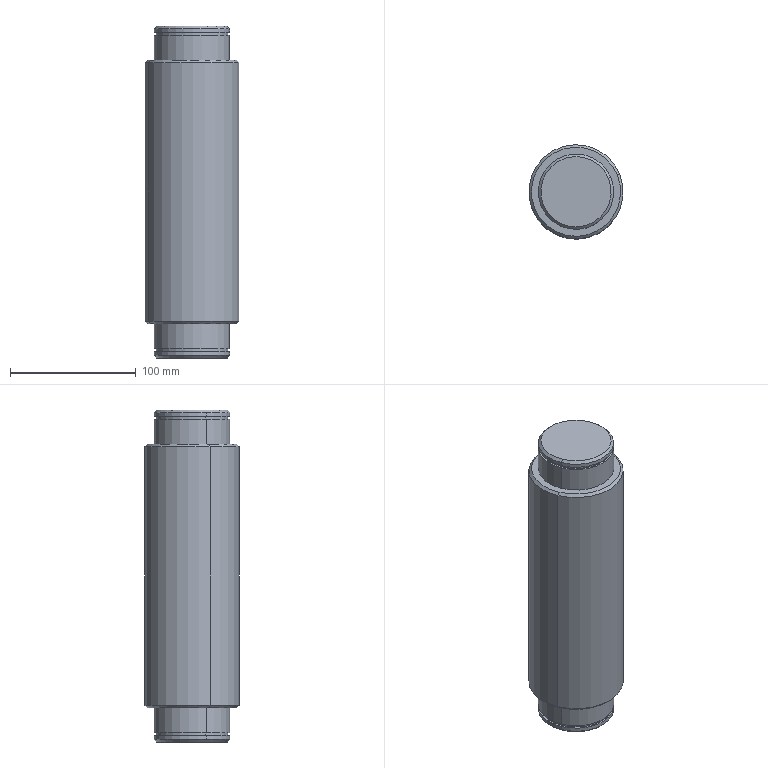Component | SolidWorks | RotationAxisB-1 | 1 solid | 30 faces | box 75 x 75 x 264.4 mm | volume 1078688 mm3 | cylinder 14 | cone 8 | plane 8 | commonest cylinder face diameters 60 x8 57 x4 75 x2 | material Stainless Steel
build123d program:
from build123d import *

# Parameters (mm, degrees)
CHAMFER1_SIZE = 2


with BuildPart() as part:
    # Sketch1 → Revolve1 (revolve)
    with BuildSketch(Plane.XY, mode=Mode.PRIVATE) as revolve1_sk:
        Polygon((0, 0), (0, 30), (5, 30), (5, 28.5), (7.2, 28.5), (7.2, 30), (27.2, 30), (27.2, 37.5), (237.2, 37.5), (237.2, 30), (257.2, 30), (257.2, 28.5), (259.4, 28.5), (259.4, 30), (264.4, 30), (264.4, 0), align=None)
    revolve(revolve1_sk.sketch.rotate(Axis((0, 0, 0), (1, 0, 0)), 90), axis=Axis((0, 0, 0), (1, 0, 0)))

    # Chamfer1
    chamfer1_edges = [part.edges().sort_by_distance(p)[0] for p in [
        (264.4, 0, -30),
        (237.2, 0, -37.5),
        (27.2, 0, -37.5),
        (0, 0, -30),
    ]]
    chamfer(chamfer1_edges, length=CHAMFER1_SIZE)


solid = part.part

# Placed as in the assembly
solid = solid.moved(Location((-534.67, 967.452, 382.9), (0, 90, 0)))
STEP:
#1=COLOUR_RGB('',0.7922,0.8196,0.9333);
#2=FILL_AREA_STYLE_COLOUR('',#1);
#3=FILL_AREA_STYLE('',(#2));
#4=SURFACE_STYLE_FILL_AREA(#3);
#5=SURFACE_SIDE_STYLE('',(#4));
#6=SURFACE_STYLE_USAGE(.BOTH.,#5);
#7=PRESENTATION_STYLE_ASSIGNMENT((#6));
#8=CARTESIAN_POINT('',(-22.068,37.666,15.075));
#9=VERTEX_POINT('',#8);
#10=CARTESIAN_POINT('',(-20.032,38.511,15.075));
#11=VERTEX_POINT('',#10);
#12=CARTESIAN_POINT('',(-21.05,38.089,15.075));
#13=DIRECTION('',(-0.,0.,1.));
#14=DIRECTION('',(0.9237,0.383,0.));
#15=AXIS2_PLACEMENT_3D('',#12,#13,#14);
#16=CIRCLE('',#15,1.102);
#17=EDGE_CURVE('',#9,#11,#16,.T.);
#18=ORIENTED_EDGE('',*,*,#17,.F.);
#19=CARTESIAN_POINT('',(-22.141,37.636,14.996));
#20=VERTEX_POINT('',#19);
#21=CARTESIAN_POINT('',(-22.068,37.666,15.075));
#22=DIRECTION('',(-0.6532,-0.2709,-0.7071));
#23=VECTOR('',#22,39.37);
#24=LINE('',#21,#23);
#25=EDGE_CURVE('',#9,#20,#24,.T.);
#26=ORIENTED_EDGE('',*,*,#25,.T.);
#27=CARTESIAN_POINT('',(-19.959,38.541,14.996));
#28=VERTEX_POINT('',#27);
#29=CARTESIAN_POINT('',(-21.05,38.089,14.996));
#30=DIRECTION('',(0.,-0.,-1.));
#31=DIRECTION('',(0.9237,0.383,0.));
#32=AXIS2_PLACEMENT_3D('',#29,#30,#31);
#33=CIRCLE('',#32,1.181);
#34=EDGE_CURVE('',#28,#20,#33,.T.);
#35=ORIENTED_EDGE('',*,*,#34,.F.);
#36=CARTESIAN_POINT('',(-20.032,38.511,15.075));
#37=DIRECTION('',(0.6532,0.2709,-0.7071));
#38=VECTOR('',#37,39.37);
#39=LINE('',#36,#38);
#40=EDGE_CURVE('',#11,#28,#39,.T.);
#41=ORIENTED_EDGE('',*,*,#40,.F.);
#42=EDGE_LOOP('',(#18,#26,#35,#41));
#43=FACE_OUTER_BOUND('',#42,.T.);
#44=CARTESIAN_POINT('',(-21.05,38.089,15.075));
#45=DIRECTION('',(0.,-0.,-1.));
#46=DIRECTION('',(0.9237,0.383,0.));
#47=AXIS2_PLACEMENT_3D('',#44,#45,#46);
#48=CONICAL_SURFACE('',#47,1.102,0.7854);
#49=ADVANCED_FACE('',(#43),#48,.T.);
#50=CARTESIAN_POINT('',(-22.341,37.553,14.004));
#51=VERTEX_POINT('',#50);
#52=CARTESIAN_POINT('',(-19.759,38.624,14.004));
#53=VERTEX_POINT('',#52);
#54=CARTESIAN_POINT('',(-21.05,38.089,14.004));
#55=DIRECTION('',(-0.,0.,1.));
#56=DIRECTION('',(0.9237,0.383,0.));
#57=AXIS2_PLACEMENT_3D('',#54,#55,#56);
#58=CIRCLE('',#57,1.398);
#59=EDGE_CURVE('',#51,#53,#58,.T.);
#60=ORIENTED_EDGE('',*,*,#59,.F.);
#61=CARTESIAN_POINT('',(-22.414,37.523,13.925));
#62=VERTEX_POINT('',#61);
#63=CARTESIAN_POINT('',(-22.341,37.553,14.004));
#64=DIRECTION('',(-0.6532,-0.2709,-0.7071));
#65=VECTOR('',#64,39.37);
#66=LINE('',#63,#65);
#67=EDGE_CURVE('',#51,#62,#66,.T.);
#68=ORIENTED_EDGE('',*,*,#67,.T.);
#69=CARTESIAN_POINT('',(-19.686,38.654,13.925));
#70=VERTEX_POINT('',#69);
#71=CARTESIAN_POINT('',(-21.05,38.089,13.925));
#72=DIRECTION('',(0.,-0.,-1.));
#73=DIRECTION('',(0.9237,0.383,0.));
#74=AXIS2_PLACEMENT_3D('',#71,#72,#73);
#75=CIRCLE('',#74,1.476);
#76=EDGE_CURVE('',#70,#62,#75,.T.);
#77=ORIENTED_EDGE('',*,*,#76,.F.);
#78=CARTESIAN_POINT('',(-19.759,38.624,14.004));
#79=DIRECTION('',(0.6532,0.2709,-0.7071));
#80=VECTOR('',#79,39.37);
#81=LINE('',#78,#80);
#82=EDGE_CURVE('',#53,#70,#81,.T.);
#83=ORIENTED_EDGE('',*,*,#82,.F.);
#84=EDGE_LOOP('',(#60,#68,#77,#83));
#85=FACE_OUTER_BOUND('',#84,.T.);
#86=CARTESIAN_POINT('',(-21.05,38.089,14.004));
#87=DIRECTION('',(0.,-0.,-1.));
#88=DIRECTION('',(0.9237,0.383,0.));
#89=AXIS2_PLACEMENT_3D('',#86,#87,#88);
#90=CONICAL_SURFACE('',#89,1.398,0.7854);
#91=ADVANCED_FACE('',(#85),#90,.T.);
#92=CARTESIAN_POINT('',(-19.759,38.624,5.736));
#93=VERTEX_POINT('',#92);
#94=CARTESIAN_POINT('',(-22.341,37.553,5.736));
#95=VERTEX_POINT('',#94);
#96=CARTESIAN_POINT('',(-21.05,38.089,5.736));
#97=DIRECTION('',(0.,-0.,-1.));
#98=DIRECTION('',(-0.9237,-0.383,0.));
#99=AXIS2_PLACEMENT_3D('',#96,#97,#98);
#100=CIRCLE('',#99,1.398);
#101=EDGE_CURVE('',#93,#95,#100,.T.);
#102=ORIENTED_EDGE('',*,*,#101,.F.);
#103=CARTESIAN_POINT('',(-19.686,38.654,5.815));
#104=VERTEX_POINT('',#103);
#105=CARTESIAN_POINT('',(-19.686,38.654,5.815));
#106=DIRECTION('',(0.6532,0.2709,0.7071));
#107=VECTOR('',#106,39.37);
#108=LINE('',#105,#107);
#109=EDGE_CURVE('',#93,#104,#108,.T.);
#110=ORIENTED_EDGE('',*,*,#109,.T.);
#111=CARTESIAN_POINT('',(-22.414,37.523,5.815));
#112=VERTEX_POINT('',#111);
#113=CARTESIAN_POINT('',(-21.05,38.089,5.815));
#114=DIRECTION('',(-0.,0.,1.));
#115=DIRECTION('',(-0.9237,-0.383,0.));
#116=AXIS2_PLACEMENT_3D('',#113,#114,#115);
#117=CIRCLE('',#116,1.476);
#118=EDGE_CURVE('',#112,#104,#117,.T.);
#119=ORIENTED_EDGE('',*,*,#118,.F.);
#120=CARTESIAN_POINT('',(-22.414,37.523,5.815));
#121=DIRECTION('',(-0.6532,-0.2709,0.7071));
#122=VECTOR('',#121,39.37);
#123=LINE('',#120,#122);
#124=EDGE_CURVE('',#95,#112,#123,.T.);
#125=ORIENTED_EDGE('',*,*,#124,.F.);
#126=EDGE_LOOP('',(#102,#110,#119,#125));
#127=FACE_OUTER_BOUND('',#126,.T.);
#128=CARTESIAN_POINT('',(-21.05,38.089,5.815));
#129=DIRECTION('',(-0.,0.,1.));
#130=DIRECTION('',(-0.9237,-0.383,0.));
#131=AXIS2_PLACEMENT_3D('',#128,#129,#130);
#132=CONICAL_SURFACE('',#131,1.476,0.7854);
#133=ADVANCED_FACE('',(#127),#132,.T.);
#134=CARTESIAN_POINT('',(-20.032,38.511,4.665));
#135=VERTEX_POINT('',#134);
#136=CARTESIAN_POINT('',(-22.068,37.666,4.665));
#137=VERTEX_POINT('',#136);
#138=CARTESIAN_POINT('',(-21.05,38.089,4.665));
#139=DIRECTION('',(0.,-0.,-1.));
#140=DIRECTION('',(-0.9237,-0.383,0.));
#141=AXIS2_PLACEMENT_3D('',#138,#139,#140);
#142=CIRCLE('',#141,1.102);
#143=EDGE_CURVE('',#135,#137,#142,.T.);
#144=ORIENTED_EDGE('',*,*,#143,.F.);
#145=CARTESIAN_POINT('',(-19.959,38.541,4.744));
#146=VERTEX_POINT('',#145);
#147=CARTESIAN_POINT('',(-19.959,38.541,4.744));
#148=DIRECTION('',(0.6532,0.2709,0.7071));
#149=VECTOR('',#148,39.37);
#150=LINE('',#147,#149);
#151=EDGE_CURVE('',#135,#146,#150,.T.);
#152=ORIENTED_EDGE('',*,*,#151,.T.);
#153=CARTESIAN_POINT('',(-22.141,37.636,4.744));
#154=VERTEX_POINT('',#153);
#155=CARTESIAN_POINT('',(-21.05,38.089,4.744));
#156=DIRECTION('',(-0.,0.,1.));
#157=DIRECTION('',(-0.9237,-0.383,0.));
#158=AXIS2_PLACEMENT_3D('',#155,#156,#157);
#159=CIRCLE('',#158,1.181);
#160=EDGE_CURVE('',#154,#146,#159,.T.);
#161=ORIENTED_EDGE('',*,*,#160,.F.);
#162=CARTESIAN_POINT('',(-22.141,37.636,4.744));
#163=DIRECTION('',(-0.6532,-0.2709,0.7071));
#164=VECTOR('',#163,39.37);
#165=LINE('',#162,#164);
#166=EDGE_CURVE('',#137,#154,#165,.T.);
#167=ORIENTED_EDGE('',*,*,#166,.F.);
#168=EDGE_LOOP('',(#144,#152,#161,#167));
#169=FACE_OUTER_BOUND('',#168,.T.);
#170=CARTESIAN_POINT('',(-21.05,38.089,4.744));
#171=DIRECTION('',(-0.,0.,1.));
#172=DIRECTION('',(-0.9237,-0.383,0.));
#173=AXIS2_PLACEMENT_3D('',#170,#171,#172);
#174=CONICAL_SURFACE('',#173,1.181,0.7854);
#175=ADVANCED_FACE('',(#169),#174,.T.);
#176=ORIENTED_EDGE('',*,*,#160,.T.);
#177=CARTESIAN_POINT('',(-19.959,38.541,4.862));
#178=VERTEX_POINT('',#177);
#179=CARTESIAN_POINT('',(-19.959,38.541,15.075));
#180=DIRECTION('',(-0.,0.,1.));
#181=VECTOR('',#180,39.37);
#182=LINE('',#179,#181);
#183=EDGE_CURVE('',#146,#178,#182,.T.);
#184=ORIENTED_EDGE('',*,*,#183,.T.);
#185=CARTESIAN_POINT('',(-22.141,37.636,4.862));
#186=VERTEX_POINT('',#185);
#187=CARTESIAN_POINT('',(-21.05,38.089,4.862));
#188=DIRECTION('',(-0.,0.,1.));
#189=DIRECTION('',(-0.9237,-0.383,0.));
#190=AXIS2_PLACEMENT_3D('',#187,#188,#189);
#191=CIRCLE('',#190,1.181);
#192=EDGE_CURVE('',#186,#178,#191,.T.);
#193=ORIENTED_EDGE('',*,*,#192,.F.);
#194=CARTESIAN_POINT('',(-22.141,37.636,15.075));
#195=DIRECTION('',(-0.,0.,1.));
#196=VECTOR('',#195,39.37);
#197=LINE('',#194,#196);
#198=EDGE_CURVE('',#154,#186,#197,.T.);
#199=ORIENTED_EDGE('',*,*,#198,.F.);
#200=EDGE_LOOP('',(#176,#184,#193,#199));
#201=FACE_OUTER_BOUND('',#200,.T.);
#202=CARTESIAN_POINT('',(-21.05,38.089,15.075));
#203=DIRECTION('',(-0.,0.,1.));
#204=DIRECTION('',(-0.9237,-0.383,0.));
#205=AXIS2_PLACEMENT_3D('',#202,#203,#204);
#206=CYLINDRICAL_SURFACE('',#205,1.181);
#207=ADVANCED_FACE('',(#201),#206,.T.);
#208=CARTESIAN_POINT('',(-22.086,37.659,4.862));
#209=VERTEX_POINT('',#208);
#210=CARTESIAN_POINT('',(-20.014,38.518,4.862));
#211=VERTEX_POINT('',#210);
#212=CARTESIAN_POINT('',(-21.05,38.089,4.862));
#213=DIRECTION('',(-0.,0.,1.));
#214=DIRECTION('',(-0.9237,-0.383,0.));
#215=AXIS2_PLACEMENT_3D('',#212,#213,#214);
#216=CIRCLE('',#215,1.122);
#217=EDGE_CURVE('',#209,#211,#216,.T.);
#218=ORIENTED_EDGE('',*,*,#217,.T.);
#219=CARTESIAN_POINT('',(-20.014,38.518,4.949));
#220=VERTEX_POINT('',#219);
#221=CARTESIAN_POINT('',(-20.014,38.518,15.075));
#222=DIRECTION('',(-0.,0.,1.));
#223=VECTOR('',#222,39.37);
#224=LINE('',#221,#223);
#225=EDGE_CURVE('',#211,#220,#224,.T.);
#226=ORIENTED_EDGE('',*,*,#225,.T.);
#227=CARTESIAN_POINT('',(-22.086,37.659,4.949));
#228=VERTEX_POINT('',#227);
#229=CARTESIAN_POINT('',(-21.05,38.089,4.949));
#230=DIRECTION('',(-0.,0.,1.));
#231=DIRECTION('',(-0.9237,-0.383,0.));
#232=AXIS2_PLACEMENT_3D('',#229,#230,#231);
#233=CIRCLE('',#232,1.122);
#234=EDGE_CURVE('',#228,#220,#233,.T.);
#235=ORIENTED_EDGE('',*,*,#234,.F.);
#236=CARTESIAN_POINT('',(-22.086,37.659,15.075));
#237=DIRECTION('',(-0.,0.,1.));
#238=VECTOR('',#237,39.37);
#239=LINE('',#236,#238);
#240=EDGE_CURVE('',#209,#228,#239,.T.);
#241=ORIENTED_EDGE('',*,*,#240,.F.);
#242=EDGE_LOOP('',(#218,#226,#235,#241));
#243=FACE_OUTER_BOUND('',#242,.T.);
#244=CARTESIAN_POINT('',(-21.05,38.089,15.075));
#245=DIRECTION('',(-0.,0.,1.));
#246=DIRECTION('',(-0.9237,-0.383,0.));
#247=AXIS2_PLACEMENT_3D('',#244,#245,#246);
#248=CYLINDRICAL_SURFACE('',#247,1.122);
#249=ADVANCED_FACE('',(#243),#248,.T.);
#250=CARTESIAN_POINT('',(-22.141,37.636,4.949));
#251=VERTEX_POINT('',#250);
#252=CARTESIAN_POINT('',(-19.959,38.541,4.949));
#253=VERTEX_POINT('',#252);
#254=CARTESIAN_POINT('',(-21.05,38.089,4.949));
#255=DIRECTION('',(-0.,0.,1.));
#256=DIRECTION('',(-0.9237,-0.383,0.));
#257=AXIS2_PLACEMENT_3D('',#254,#255,#256);
#258=CIRCLE('',#257,1.181);
#259=EDGE_CURVE('',#251,#253,#258,.T.);
#260=ORIENTED_EDGE('',*,*,#259,.T.);
#261=CARTESIAN_POINT('',(-19.959,38.541,5.736));
#262=VERTEX_POINT('',#261);
#263=CARTESIAN_POINT('',(-19.959,38.541,15.075));
#264=DIRECTION('',(-0.,0.,1.));
#265=VECTOR('',#264,39.37);
#266=LINE('',#263,#265);
#267=EDGE_CURVE('',#253,#262,#266,.T.);
#268=ORIENTED_EDGE('',*,*,#267,.T.);
#269=CARTESIAN_POINT('',(-22.141,37.636,5.736));
#270=VERTEX_POINT('',#269);
#271=CARTESIAN_POINT('',(-21.05,38.089,5.736));
#272=DIRECTION('',(-0.,0.,1.));
#273=DIRECTION('',(-0.9237,-0.383,0.));
#274=AXIS2_PLACEMENT_3D('',#271,#272,#273);
#275=CIRCLE('',#274,1.181);
#276=EDGE_CURVE('',#270,#262,#275,.T.);
#277=ORIENTED_EDGE('',*,*,#276,.F.);
#278=CARTESIAN_POINT('',(-22.141,37.636,15.075));
#279=DIRECTION('',(-0.,0.,1.));
#280=VECTOR('',#279,39.37);
#281=LINE('',#278,#280);
#282=EDGE_CURVE('',#251,#270,#281,.T.);
#283=ORIENTED_EDGE('',*,*,#282,.F.);
#284=EDGE_LOOP('',(#260,#268,#277,#283));
#285=FACE_OUTER_BOUND('',#284,.T.);
#286=CARTESIAN_POINT('',(-21.05,38.089,15.075));
#287=DIRECTION('',(-0.,0.,1.));
#288=DIRECTION('',(-0.9237,-0.383,0.));
#289=AXIS2_PLACEMENT_3D('',#286,#287,#288);
#290=CYLINDRICAL_SURFACE('',#289,1.181);
#291=ADVANCED_FACE('',(#285),#290,.T.);
#292=ORIENTED_EDGE('',*,*,#118,.T.);
#293=CARTESIAN_POINT('',(-19.686,38.654,15.075));
#294=DIRECTION('',(-0.,0.,1.));
#295=VECTOR('',#294,39.37);
#296=LINE('',#293,#295);
#297=EDGE_CURVE('',#104,#70,#296,.T.);
#298=ORIENTED_EDGE('',*,*,#297,.T.);
#299=ORIENTED_EDGE('',*,*,#76,.T.);
#300=CARTESIAN_POINT('',(-22.414,37.523,15.075));
#301=DIRECTION('',(-0.,0.,1.));
#302=VECTOR('',#301,39.37);
#303=LINE('',#300,#302);
#304=EDGE_CURVE('',#112,#62,#303,.T.);
#305=ORIENTED_EDGE('',*,*,#304,.F.);
#306=EDGE_LOOP('',(#292,#298,#299,#305));
#307=FACE_OUTER_BOUND('',#306,.T.);
#308=CARTESIAN_POINT('',(-21.05,38.089,15.075));
#309=DIRECTION('',(-0.,0.,1.));
#310=DIRECTION('',(-0.9237,-0.383,0.));
#311=AXIS2_PLACEMENT_3D('',#308,#309,#310);
#312=CYLINDRICAL_SURFACE('',#311,1.476);
#313=ADVANCED_FACE('',(#307),#312,.T.);
#314=CARTESIAN_POINT('',(-22.141,37.636,14.004));
#315=VERTEX_POINT('',#314);
#316=CARTESIAN_POINT('',(-19.959,38.541,14.004));
#317=VERTEX_POINT('',#316);
#318=CARTESIAN_POINT('',(-21.05,38.089,14.004));
#319=DIRECTION('',(-0.,0.,1.));
#320=DIRECTION('',(-0.9237,-0.383,0.));
#321=AXIS2_PLACEMENT_3D('',#318,#319,#320);
#322=CIRCLE('',#321,1.181);
#323=EDGE_CURVE('',#315,#317,#322,.T.);
#324=ORIENTED_EDGE('',*,*,#323,.T.);
#325=CARTESIAN_POINT('',(-19.959,38.541,14.791));
#326=VERTEX_POINT('',#325);
#327=CARTESIAN_POINT('',(-19.959,38.541,15.075));
#328=DIRECTION('',(-0.,0.,1.));
#329=VECTOR('',#328,39.37);
#330=LINE('',#327,#329);
#331=EDGE_CURVE('',#317,#326,#330,.T.);
#332=ORIENTED_EDGE('',*,*,#331,.T.);
#333=CARTESIAN_POINT('',(-22.141,37.636,14.791));
#334=VERTEX_POINT('',#333);
#335=CARTESIAN_POINT('',(-21.05,38.089,14.791));
#336=DIRECTION('',(-0.,0.,1.));
#337=DIRECTION('',(-0.9237,-0.383,0.));
#338=AXIS2_PLACEMENT_3D('',#335,#336,#337);
#339=CIRCLE('',#338,1.181);
#340=EDGE_CURVE('',#334,#326,#339,.T.);
#341=ORIENTED_EDGE('',*,*,#340,.F.);
#342=CARTESIAN_POINT('',(-22.141,37.636,15.075));
#343=DIRECTION('',(-0.,0.,1.));
#344=VECTOR('',#343,39.37);
#345=LINE('',#342,#344);
#346=EDGE_CURVE('',#315,#334,#345,.T.);
#347=ORIENTED_EDGE('',*,*,#346,.F.);
#348=EDGE_LOOP('',(#324,#332,#341,#347));
#349=FACE_OUTER_BOUND('',#348,.T.);
#350=CARTESIAN_POINT('',(-21.05,38.089,15.075));
#351=DIRECTION('',(-0.,0.,1.));
#352=DIRECTION('',(-0.9237,-0.383,0.));
#353=AXIS2_PLACEMENT_3D('',#350,#351,#352);
#354=CYLINDRICAL_SURFACE('',#353,1.181);
#355=ADVANCED_FACE('',(#349),#354,.T.);
#356=CARTESIAN_POINT('',(-22.086,37.659,14.791));
#357=VERTEX_POINT('',#356);
#358=CARTESIAN_POINT('',(-20.014,38.518,14.791));
#359=VERTEX_POINT('',#358);
#360=CARTESIAN_POINT('',(-21.05,38.089,14.791));
#361=DIRECTION('',(-0.,0.,1.));
#362=DIRECTION('',(-0.9237,-0.383,0.));
#363=AXIS2_PLACEMENT_3D('',#360,#361,#362);
#364=CIRCLE('',#363,1.122);
#365=EDGE_CURVE('',#357,#359,#364,.T.);
#366=ORIENTED_EDGE('',*,*,#365,.T.);
#367=CARTESIAN_POINT('',(-20.014,38.518,14.878));
#368=VERTEX_POINT('',#367);
#369=CARTESIAN_POINT('',(-20.014,38.518,15.075));
#370=DIRECTION('',(-0.,0.,1.));
#371=VECTOR('',#370,39.37);
#372=LINE('',#369,#371);
#373=EDGE_CURVE('',#359,#368,#372,.T.);
#374=ORIENTED_EDGE('',*,*,#373,.T.);
#375=CARTESIAN_POINT('',(-22.086,37.659,14.878));
#376=VERTEX_POINT('',#375);
#377=CARTESIAN_POINT('',(-21.05,38.089,14.878));
#378=DIRECTION('',(-0.,0.,1.));
#379=DIRECTION('',(-0.9237,-0.383,0.));
#380=AXIS2_PLACEMENT_3D('',#377,#378,#379);
#381=CIRCLE('',#380,1.122);
#382=EDGE_CURVE('',#376,#368,#381,.T.);
#383=ORIENTED_EDGE('',*,*,#382,.F.);
#384=CARTESIAN_POINT('',(-22.086,37.659,15.075));
#385=DIRECTION('',(-0.,0.,1.));
#386=VECTOR('',#385,39.37);
#387=LINE('',#384,#386);
#388=EDGE_CURVE('',#357,#376,#387,.T.);
#389=ORIENTED_EDGE('',*,*,#388,.F.);
#390=EDGE_LOOP('',(#366,#374,#383,#389));
#391=FACE_OUTER_BOUND('',#390,.T.);
#392=CARTESIAN_POINT('',(-21.05,38.089,15.075));
#393=DIRECTION('',(-0.,0.,1.));
#394=DIRECTION('',(-0.9237,-0.383,0.));
#395=AXIS2_PLACEMENT_3D('',#392,#393,#394);
#396=CYLINDRICAL_SURFACE('',#395,1.122);
#397=ADVANCED_FACE('',(#391),#396,.T.);
#398=CARTESIAN_POINT('',(-22.141,37.636,14.878));
#399=VERTEX_POINT('',#398);
#400=CARTESIAN_POINT('',(-19.959,38.541,14.878));
#401=VERTEX_POINT('',#400);
#402=CARTESIAN_POINT('',(-21.05,38.089,14.878));
#403=DIRECTION('',(-0.,0.,1.));
#404=DIRECTION('',(-0.9237,-0.383,0.));
#405=AXIS2_PLACEMENT_3D('',#402,#403,#404);
#406=CIRCLE('',#405,1.181);
#407=EDGE_CURVE('',#399,#401,#406,.T.);
#408=ORIENTED_EDGE('',*,*,#407,.T.);
#409=CARTESIAN_POINT('',(-19.959,38.541,15.075));
#410=DIRECTION('',(-0.,0.,1.));
#411=VECTOR('',#410,39.37);
#412=LINE('',#409,#411);
#413=EDGE_CURVE('',#401,#28,#412,.T.);
#414=ORIENTED_EDGE('',*,*,#413,.T.);
#415=ORIENTED_EDGE('',*,*,#34,.T.);
#416=CARTESIAN_POINT('',(-22.141,37.636,15.075));
#417=DIRECTION('',(-0.,0.,1.));
#418=VECTOR('',#417,39.37);
#419=LINE('',#416,#418);
#420=EDGE_CURVE('',#399,#20,#419,.T.);
#421=ORIENTED_EDGE('',*,*,#420,.F.);
#422=EDGE_LOOP('',(#408,#414,#415,#421));
#423=FACE_OUTER_BOUND('',#422,.T.);
#424=CARTESIAN_POINT('',(-21.05,38.089,15.075));
#425=DIRECTION('',(-0.,0.,1.));
#426=DIRECTION('',(-0.9237,-0.383,0.));
#427=AXIS2_PLACEMENT_3D('',#424,#425,#426);
#428=CYLINDRICAL_SURFACE('',#427,1.181);
#429=ADVANCED_FACE('',(#423),#428,.T.);
#430=CARTESIAN_POINT('',(-21.05,38.089,15.075));
#431=DIRECTION('',(-0.,0.,1.));
#432=DIRECTION('',(0.9237,0.383,0.));
#433=AXIS2_PLACEMENT_3D('',#430,#431,#432);
#434=CIRCLE('',#433,1.102);
#435=EDGE_CURVE('',#11,#9,#434,.T.);
#436=ORIENTED_EDGE('',*,*,#435,.T.);
#437=ORIENTED_EDGE('',*,*,#17,.T.);
#438=EDGE_LOOP('',(#436,#437));
#439=FACE_OUTER_BOUND('',#438,.T.);
#440=CARTESIAN_POINT('',(-21.05,38.089,15.075));
#441=DIRECTION('',(0.,-0.,-1.));
#442=DIRECTION('',(0.9237,0.383,0.));
#443=AXIS2_PLACEMENT_3D('',#440,#441,#442);
#444=PLANE('',#443);
#445=ADVANCED_FACE('',(#439),#444,.F.);
#446=ORIENTED_EDGE('',*,*,#413,.F.);
#447=CARTESIAN_POINT('',(-21.05,38.089,14.878));
#448=DIRECTION('',(-0.,0.,1.));
#449=DIRECTION('',(-0.9237,-0.383,0.));
#450=AXIS2_PLACEMENT_3D('',#447,#448,#449);
#451=CIRCLE('',#450,1.181);
#452=EDGE_CURVE('',#401,#399,#451,.T.);
#453=ORIENTED_EDGE('',*,*,#452,.T.);
#454=ORIENTED_EDGE('',*,*,#420,.T.);
#455=CARTESIAN_POINT('',(-21.05,38.089,14.996));
#456=DIRECTION('',(0.,-0.,-1.));
#457=DIRECTION('',(0.9237,0.383,0.));
#458=AXIS2_PLACEMENT_3D('',#455,#456,#457);
#459=CIRCLE('',#458,1.181);
#460=EDGE_CURVE('',#20,#28,#459,.T.);
#461=ORIENTED_EDGE('',*,*,#460,.T.);
#462=EDGE_LOOP('',(#446,#453,#454,#461));
#463=FACE_OUTER_BOUND('',#462,.T.);
#464=CARTESIAN_POINT('',(-21.05,38.089,15.075));
#465=DIRECTION('',(-0.,0.,1.));
#466=DIRECTION('',(-0.9237,-0.383,0.));
#467=AXIS2_PLACEMENT_3D('',#464,#465,#466);
#468=CYLINDRICAL_SURFACE('',#467,1.181);
#469=ADVANCED_FACE('',(#463),#468,.T.);
#470=ORIENTED_EDGE('',*,*,#407,.F.);
#471=ORIENTED_EDGE('',*,*,#452,.F.);
#472=EDGE_LOOP('',(#470,#471));
#473=FACE_OUTER_BOUND('',#472,.T.);
#474=ORIENTED_EDGE('',*,*,#382,.T.);
#475=CARTESIAN_POINT('',(-21.05,38.089,14.878));
#476=DIRECTION('',(-0.,0.,1.));
#477=DIRECTION('',(-0.9237,-0.383,0.));
#478=AXIS2_PLACEMENT_3D('',#475,#476,#477);
#479=CIRCLE('',#478,1.122);
#480=EDGE_CURVE('',#368,#376,#479,.T.);
#481=ORIENTED_EDGE('',*,*,#480,.T.);
#482=EDGE_LOOP('',(#474,#481));
#483=FACE_BOUND('',#482,.T.);
#484=CARTESIAN_POINT('',(-20.598,36.998,14.878));
#485=DIRECTION('',(-0.,0.,1.));
#486=DIRECTION('',(-0.9237,-0.383,-0.));
#487=AXIS2_PLACEMENT_3D('',#484,#485,#486);
#488=PLANE('',#487);
#489=ADVANCED_FACE('',(#473,#483),#488,.F.);
#490=ORIENTED_EDGE('',*,*,#373,.F.);
#491=CARTESIAN_POINT('',(-21.05,38.089,14.791));
#492=DIRECTION('',(-0.,0.,1.));
#493=DIRECTION('',(-0.9237,-0.383,0.));
#494=AXIS2_PLACEMENT_3D('',#491,#492,#493);
#495=CIRCLE('',#494,1.122);
#496=EDGE_CURVE('',#359,#357,#495,.T.);
#497=ORIENTED_EDGE('',*,*,#496,.T.);
#498=ORIENTED_EDGE('',*,*,#388,.T.);
#499=ORIENTED_EDGE('',*,*,#480,.F.);
#500=EDGE_LOOP('',(#490,#497,#498,#499));
#501=FACE_OUTER_BOUND('',#500,.T.);
#502=CARTESIAN_POINT('',(-21.05,38.089,15.075));
#503=DIRECTION('',(-0.,0.,1.));
#504=DIRECTION('',(-0.9237,-0.383,0.));
#505=AXIS2_PLACEMENT_3D('',#502,#503,#504);
#506=CYLINDRICAL_SURFACE('',#505,1.122);
#507=ADVANCED_FACE('',(#501),#506,.T.);
#508=ORIENTED_EDGE('',*,*,#365,.F.);
#509=ORIENTED_EDGE('',*,*,#496,.F.);
#510=EDGE_LOOP('',(#508,#509));
#511=FACE_BOUND('',#510,.T.);
#512=ORIENTED_EDGE('',*,*,#340,.T.);
#513=CARTESIAN_POINT('',(-21.05,38.089,14.791));
#514=DIRECTION('',(-0.,0.,1.));
#515=DIRECTION('',(-0.9237,-0.383,0.));
#516=AXIS2_PLACEMENT_3D('',#513,#514,#515);
#517=CIRCLE('',#516,1.181);
#518=EDGE_CURVE('',#326,#334,#517,.T.);
#519=ORIENTED_EDGE('',*,*,#518,.T.);
#520=EDGE_LOOP('',(#512,#519));
#521=FACE_OUTER_BOUND('',#520,.T.);
#522=CARTESIAN_POINT('',(-20.62,37.052,14.791));
#523=DIRECTION('',(0.,-0.,-1.));
#524=DIRECTION('',(0.9237,0.383,0.));
#525=AXIS2_PLACEMENT_3D('',#522,#523,#524);
#526=PLANE('',#525);
#527=ADVANCED_FACE('',(#511,#521),#526,.F.);
#528=ORIENTED_EDGE('',*,*,#331,.F.);
#529=CARTESIAN_POINT('',(-21.05,38.089,14.004));
#530=DIRECTION('',(-0.,0.,1.));
#531=DIRECTION('',(-0.9237,-0.383,0.));
#532=AXIS2_PLACEMENT_3D('',#529,#530,#531);
#533=CIRCLE('',#532,1.181);
#534=EDGE_CURVE('',#317,#315,#533,.T.);
#535=ORIENTED_EDGE('',*,*,#534,.T.);
#536=ORIENTED_EDGE('',*,*,#346,.T.);
#537=ORIENTED_EDGE('',*,*,#518,.F.);
#538=EDGE_LOOP('',(#528,#535,#536,#537));
#539=FACE_OUTER_BOUND('',#538,.T.);
#540=CARTESIAN_POINT('',(-21.05,38.089,15.075));
#541=DIRECTION('',(-0.,0.,1.));
#542=DIRECTION('',(-0.9237,-0.383,0.));
#543=AXIS2_PLACEMENT_3D('',#540,#541,#542);
#544=CYLINDRICAL_SURFACE('',#543,1.181);
#545=ADVANCED_FACE('',(#539),#544,.T.);
#546=CARTESIAN_POINT('',(-21.05,38.089,14.004));
#547=DIRECTION('',(-0.,0.,1.));
#548=DIRECTION('',(0.9237,0.383,0.));
#549=AXIS2_PLACEMENT_3D('',#546,#547,#548);
#550=CIRCLE('',#549,1.398);
#551=EDGE_CURVE('',#53,#51,#550,.T.);
#552=ORIENTED_EDGE('',*,*,#551,.T.);
#553=ORIENTED_EDGE('',*,*,#59,.T.);
#554=EDGE_LOOP('',(#552,#553));
#555=FACE_OUTER_BOUND('',#554,.T.);
#556=ORIENTED_EDGE('',*,*,#323,.F.);
#557=ORIENTED_EDGE('',*,*,#534,.F.);
#558=EDGE_LOOP('',(#556,#557));
#559=FACE_BOUND('',#558,.T.);
#560=CARTESIAN_POINT('',(-20.598,36.998,14.004));
#561=DIRECTION('',(0.,-0.,-1.));
#562=DIRECTION('',(0.9237,0.383,0.));
#563=AXIS2_PLACEMENT_3D('',#560,#561,#562);
#564=PLANE('',#563);
#565=ADVANCED_FACE('',(#555,#559),#564,.F.);
#566=ORIENTED_EDGE('',*,*,#297,.F.);
#567=CARTESIAN_POINT('',(-21.05,38.089,5.815));
#568=DIRECTION('',(-0.,0.,1.));
#569=DIRECTION('',(-0.9237,-0.383,0.));
#570=AXIS2_PLACEMENT_3D('',#567,#568,#569);
#571=CIRCLE('',#570,1.476);
#572=EDGE_CURVE('',#104,#112,#571,.T.);
#573=ORIENTED_EDGE('',*,*,#572,.T.);
#574=ORIENTED_EDGE('',*,*,#304,.T.);
#575=CARTESIAN_POINT('',(-21.05,38.089,13.925));
#576=DIRECTION('',(0.,-0.,-1.));
#577=DIRECTION('',(0.9237,0.383,0.));
#578=AXIS2_PLACEMENT_3D('',#575,#576,#577);
#579=CIRCLE('',#578,1.476);
#580=EDGE_CURVE('',#62,#70,#579,.T.);
#581=ORIENTED_EDGE('',*,*,#580,.T.);
#582=EDGE_LOOP('',(#566,#573,#574,#581));
#583=FACE_OUTER_BOUND('',#582,.T.);
#584=CARTESIAN_POINT('',(-21.05,38.089,15.075));
#585=DIRECTION('',(-0.,0.,1.));
#586=DIRECTION('',(-0.9237,-0.383,0.));
#587=AXIS2_PLACEMENT_3D('',#584,#585,#586);
#588=CYLINDRICAL_SURFACE('',#587,1.476);
#589=ADVANCED_FACE('',(#583),#588,.T.);
#590=CARTESIAN_POINT('',(-21.05,38.089,5.736));
#591=DIRECTION('',(0.,-0.,-1.));
#592=DIRECTION('',(-0.9237,-0.383,0.));
#593=AXIS2_PLACEMENT_3D('',#590,#591,#592);
#594=CIRCLE('',#593,1.398);
#595=EDGE_CURVE('',#95,#93,#594,.T.);
#596=ORIENTED_EDGE('',*,*,#595,.T.);
#597=ORIENTED_EDGE('',*,*,#101,.T.);
#598=EDGE_LOOP('',(#596,#597));
#599=FACE_OUTER_BOUND('',#598,.T.);
#600=ORIENTED_EDGE('',*,*,#276,.T.);
#601=CARTESIAN_POINT('',(-21.05,38.089,5.736));
#602=DIRECTION('',(-0.,0.,1.));
#603=DIRECTION('',(-0.9237,-0.383,0.));
#604=AXIS2_PLACEMENT_3D('',#601,#602,#603);
#605=CIRCLE('',#604,1.181);
#606=EDGE_CURVE('',#262,#270,#605,.T.);
#607=ORIENTED_EDGE('',*,*,#606,.T.);
#608=EDGE_LOOP('',(#600,#607));
#609=FACE_BOUND('',#608,.T.);
#610=CARTESIAN_POINT('',(-20.484,36.725,5.736));
#611=DIRECTION('',(-0.,0.,1.));
#612=DIRECTION('',(-0.9237,-0.383,-0.));
#613=AXIS2_PLACEMENT_3D('',#610,#611,#612);
#614=PLANE('',#613);
#615=ADVANCED_FACE('',(#599,#609),#614,.F.);
#616=ORIENTED_EDGE('',*,*,#267,.F.);
#617=CARTESIAN_POINT('',(-21.05,38.089,4.949));
#618=DIRECTION('',(-0.,0.,1.));
#619=DIRECTION('',(-0.9237,-0.383,0.));
#620=AXIS2_PLACEMENT_3D('',#617,#618,#619);
#621=CIRCLE('',#620,1.181);
#622=EDGE_CURVE('',#253,#251,#621,.T.);
#623=ORIENTED_EDGE('',*,*,#622,.T.);
#624=ORIENTED_EDGE('',*,*,#282,.T.);
#625=ORIENTED_EDGE('',*,*,#606,.F.);
#626=EDGE_LOOP('',(#616,#623,#624,#625));
#627=FACE_OUTER_BOUND('',#626,.T.);
#628=CARTESIAN_POINT('',(-21.05,38.089,15.075));
#629=DIRECTION('',(-0.,0.,1.));
#630=DIRECTION('',(-0.9237,-0.383,0.));
#631=AXIS2_PLACEMENT_3D('',#628,#629,#630);
#632=CYLINDRICAL_SURFACE('',#631,1.181);
#633=ADVANCED_FACE('',(#627),#632,.T.);
#634=ORIENTED_EDGE('',*,*,#259,.F.);
#635=ORIENTED_EDGE('',*,*,#622,.F.);
#636=EDGE_LOOP('',(#634,#635));
#637=FACE_OUTER_BOUND('',#636,.T.);
#638=ORIENTED_EDGE('',*,*,#234,.T.);
#639=CARTESIAN_POINT('',(-21.05,38.089,4.949));
#640=DIRECTION('',(-0.,0.,1.));
#641=DIRECTION('',(-0.9237,-0.383,0.));
#642=AXIS2_PLACEMENT_3D('',#639,#640,#641);
#643=CIRCLE('',#642,1.122);
#644=EDGE_CURVE('',#220,#228,#643,.T.);
#645=ORIENTED_EDGE('',*,*,#644,.T.);
#646=EDGE_LOOP('',(#638,#645));
#647=FACE_BOUND('',#646,.T.);
#648=CARTESIAN_POINT('',(-20.598,36.998,4.949));
#649=DIRECTION('',(-0.,0.,1.));
#650=DIRECTION('',(-0.9237,-0.383,-0.));
#651=AXIS2_PLACEMENT_3D('',#648,#649,#650);
#652=PLANE('',#651);
#653=ADVANCED_FACE('',(#637,#647),#652,.F.);
#654=ORIENTED_EDGE('',*,*,#225,.F.);
#655=CARTESIAN_POINT('',(-21.05,38.089,4.862));
#656=DIRECTION('',(-0.,0.,1.));
#657=DIRECTION('',(-0.9237,-0.383,0.));
#658=AXIS2_PLACEMENT_3D('',#655,#656,#657);
#659=CIRCLE('',#658,1.122);
#660=EDGE_CURVE('',#211,#209,#659,.T.);
#661=ORIENTED_EDGE('',*,*,#660,.T.);
#662=ORIENTED_EDGE('',*,*,#240,.T.);
#663=ORIENTED_EDGE('',*,*,#644,.F.);
#664=EDGE_LOOP('',(#654,#661,#662,#663));
#665=FACE_OUTER_BOUND('',#664,.T.);
#666=CARTESIAN_POINT('',(-21.05,38.089,15.075));
#667=DIRECTION('',(-0.,0.,1.));
#668=DIRECTION('',(-0.9237,-0.383,0.));
#669=AXIS2_PLACEMENT_3D('',#666,#667,#668);
#670=CYLINDRICAL_SURFACE('',#669,1.122);
#671=ADVANCED_FACE('',(#665),#670,.T.);
#672=ORIENTED_EDGE('',*,*,#217,.F.);
#673=ORIENTED_EDGE('',*,*,#660,.F.);
#674=EDGE_LOOP('',(#672,#673));
#675=FACE_BOUND('',#674,.T.);
#676=ORIENTED_EDGE('',*,*,#192,.T.);
#677=CARTESIAN_POINT('',(-21.05,38.089,4.862));
#678=DIRECTION('',(-0.,0.,1.));
#679=DIRECTION('',(-0.9237,-0.383,0.));
#680=AXIS2_PLACEMENT_3D('',#677,#678,#679);
#681=CIRCLE('',#680,1.181);
#682=EDGE_CURVE('',#178,#186,#681,.T.);
#683=ORIENTED_EDGE('',*,*,#682,.T.);
#684=EDGE_LOOP('',(#676,#683));
#685=FACE_OUTER_BOUND('',#684,.T.);
#686=CARTESIAN_POINT('',(-20.62,37.052,4.862));
#687=DIRECTION('',(0.,-0.,-1.));
#688=DIRECTION('',(0.9237,0.383,0.));
#689=AXIS2_PLACEMENT_3D('',#686,#687,#688);
#690=PLANE('',#689);
#691=ADVANCED_FACE('',(#675,#685),#690,.F.);
#692=ORIENTED_EDGE('',*,*,#183,.F.);
#693=CARTESIAN_POINT('',(-21.05,38.089,4.744));
#694=DIRECTION('',(-0.,0.,1.));
#695=DIRECTION('',(-0.9237,-0.383,0.));
#696=AXIS2_PLACEMENT_3D('',#693,#694,#695);
#697=CIRCLE('',#696,1.181);
#698=EDGE_CURVE('',#146,#154,#697,.T.);
#699=ORIENTED_EDGE('',*,*,#698,.T.);
#700=ORIENTED_EDGE('',*,*,#198,.T.);
#701=ORIENTED_EDGE('',*,*,#682,.F.);
#702=EDGE_LOOP('',(#692,#699,#700,#701));
#703=FACE_OUTER_BOUND('',#702,.T.);
#704=CARTESIAN_POINT('',(-21.05,38.089,15.075));
#705=DIRECTION('',(-0.,0.,1.));
#706=DIRECTION('',(-0.9237,-0.383,0.));
#707=AXIS2_PLACEMENT_3D('',#704,#705,#706);
#708=CYLINDRICAL_SURFACE('',#707,1.181);
#709=ADVANCED_FACE('',(#703),#708,.T.);
#710=CARTESIAN_POINT('',(-21.05,38.089,4.665));
#711=DIRECTION('',(0.,-0.,-1.));
#712=DIRECTION('',(-0.9237,-0.383,0.));
#713=AXIS2_PLACEMENT_3D('',#710,#711,#712);
#714=CIRCLE('',#713,1.102);
#715=EDGE_CURVE('',#137,#135,#714,.T.);
#716=ORIENTED_EDGE('',*,*,#715,.T.);
#717=ORIENTED_EDGE('',*,*,#143,.T.);
#718=EDGE_LOOP('',(#716,#717));
#719=FACE_OUTER_BOUND('',#718,.T.);
#720=CARTESIAN_POINT('',(-20.598,36.998,4.665));
#721=DIRECTION('',(-0.,0.,1.));
#722=DIRECTION('',(-0.9237,-0.383,-0.));
#723=AXIS2_PLACEMENT_3D('',#720,#721,#722);
#724=PLANE('',#723);
#725=ADVANCED_FACE('',(#719),#724,.F.);
#726=ORIENTED_EDGE('',*,*,#151,.F.);
#727=ORIENTED_EDGE('',*,*,#715,.F.);
#728=ORIENTED_EDGE('',*,*,#166,.T.);
#729=ORIENTED_EDGE('',*,*,#698,.F.);
#730=EDGE_LOOP('',(#726,#727,#728,#729));
#731=FACE_OUTER_BOUND('',#730,.T.);
#732=CARTESIAN_POINT('',(-21.05,38.089,4.744));
#733=DIRECTION('',(-0.,0.,1.));
#734=DIRECTION('',(-0.9237,-0.383,0.));
#735=AXIS2_PLACEMENT_3D('',#732,#733,#734);
#736=CONICAL_SURFACE('',#735,1.181,0.7854);
#737=ADVANCED_FACE('',(#731),#736,.T.);
#738=ORIENTED_EDGE('',*,*,#109,.F.);
#739=ORIENTED_EDGE('',*,*,#595,.F.);
#740=ORIENTED_EDGE('',*,*,#124,.T.);
#741=ORIENTED_EDGE('',*,*,#572,.F.);
#742=EDGE_LOOP('',(#738,#739,#740,#741));
#743=FACE_OUTER_BOUND('',#742,.T.);
#744=CARTESIAN_POINT('',(-21.05,38.089,5.815));
#745=DIRECTION('',(-0.,0.,1.));
#746=DIRECTION('',(-0.9237,-0.383,0.));
#747=AXIS2_PLACEMENT_3D('',#744,#745,#746);
#748=CONICAL_SURFACE('',#747,1.476,0.7854);
#749=ADVANCED_FACE('',(#743),#748,.T.);
#750=ORIENTED_EDGE('',*,*,#67,.F.);
#751=ORIENTED_EDGE('',*,*,#551,.F.);
#752=ORIENTED_EDGE('',*,*,#82,.T.);
#753=ORIENTED_EDGE('',*,*,#580,.F.);
#754=EDGE_LOOP('',(#750,#751,#752,#753));
#755=FACE_OUTER_BOUND('',#754,.T.);
#756=CARTESIAN_POINT('',(-21.05,38.089,14.004));
#757=DIRECTION('',(0.,-0.,-1.));
#758=DIRECTION('',(0.9237,0.383,0.));
#759=AXIS2_PLACEMENT_3D('',#756,#757,#758);
#760=CONICAL_SURFACE('',#759,1.398,0.7854);
#761=ADVANCED_FACE('',(#755),#760,.T.);
#762=ORIENTED_EDGE('',*,*,#25,.F.);
#763=ORIENTED_EDGE('',*,*,#435,.F.);
#764=ORIENTED_EDGE('',*,*,#40,.T.);
#765=ORIENTED_EDGE('',*,*,#460,.F.);
#766=EDGE_LOOP('',(#762,#763,#764,#765));
#767=FACE_OUTER_BOUND('',#766,.T.);
#768=CARTESIAN_POINT('',(-21.05,38.089,15.075));
#769=DIRECTION('',(0.,-0.,-1.));
#770=DIRECTION('',(0.9237,0.383,0.));
#771=AXIS2_PLACEMENT_3D('',#768,#769,#770);
#772=CONICAL_SURFACE('',#771,1.102,0.7854);
#773=ADVANCED_FACE('',(#767),#772,.T.);
#774=CLOSED_SHELL('',(#49,#91,#133,#175,#207,#249,#291,#313,#355,#397,#429,#445,#469,#489,#507,#527,#545,#565,#589,#615,#633,#653,#671,#691,#709,#725,#737,#749,#761,#773));
#775=MANIFOLD_SOLID_BREP('',#774);
#776=STYLED_ITEM('',(#7),#775);
#777=PRESENTATION_LAYER_ASSIGNMENT('','',(#776));
#778=(LENGTH_UNIT()NAMED_UNIT(*)SI_UNIT($,.METRE.));
#779=LENGTH_MEASURE_WITH_UNIT(LENGTH_MEASURE(0.0254),#778);
#780=DIMENSIONAL_EXPONENTS(1.,0.,0.,0.,0.,0.,0.);
#781=(CONVERSION_BASED_UNIT('',#779)LENGTH_UNIT()NAMED_UNIT(#780));
#782=UNCERTAINTY_MEASURE_WITH_UNIT(LENGTH_MEASURE(0.00001),#781,'','');
#783=(NAMED_UNIT(*)PLANE_ANGLE_UNIT()SI_UNIT($,.RADIAN.));
#784=(NAMED_UNIT(*)SI_UNIT($,.STERADIAN.)SOLID_ANGLE_UNIT());
#785=(GEOMETRIC_REPRESENTATION_CONTEXT(3)GLOBAL_UNCERTAINTY_ASSIGNED_CONTEXT((#782))GLOBAL_UNIT_ASSIGNED_CONTEXT((#781,#783,#784))REPRESENTATION_CONTEXT('',''));
#786=MECHANICAL_DESIGN_GEOMETRIC_PRESENTATION_REPRESENTATION('',(#776),#785);
#787=CARTESIAN_POINT('',(0.,0.,0.));
#788=DIRECTION('',(0.,0.,1.));
#789=DIRECTION('',(1.,0.,0.));
#790=AXIS2_PLACEMENT_3D('',#787,#788,#789);
#791=(LENGTH_UNIT()NAMED_UNIT(*)SI_UNIT($,.METRE.));
#792=LENGTH_MEASURE_WITH_UNIT(LENGTH_MEASURE(0.0254),#791);
#793=DIMENSIONAL_EXPONENTS(1.,0.,0.,0.,0.,0.,0.);
#794=(CONVERSION_BASED_UNIT('',#792)LENGTH_UNIT()NAMED_UNIT(#793));
#795=UNCERTAINTY_MEASURE_WITH_UNIT(LENGTH_MEASURE(0.00001),#794,'','');
#796=(NAMED_UNIT(*)PLANE_ANGLE_UNIT()SI_UNIT($,.RADIAN.));
#797=(NAMED_UNIT(*)SI_UNIT($,.STERADIAN.)SOLID_ANGLE_UNIT());
#798=(GEOMETRIC_REPRESENTATION_CONTEXT(3)GLOBAL_UNCERTAINTY_ASSIGNED_CONTEXT((#795))GLOBAL_UNIT_ASSIGNED_CONTEXT((#794,#796,#797))REPRESENTATION_CONTEXT('',''));
#799=ADVANCED_BREP_SHAPE_REPRESENTATION('',(#775,#790),#798);